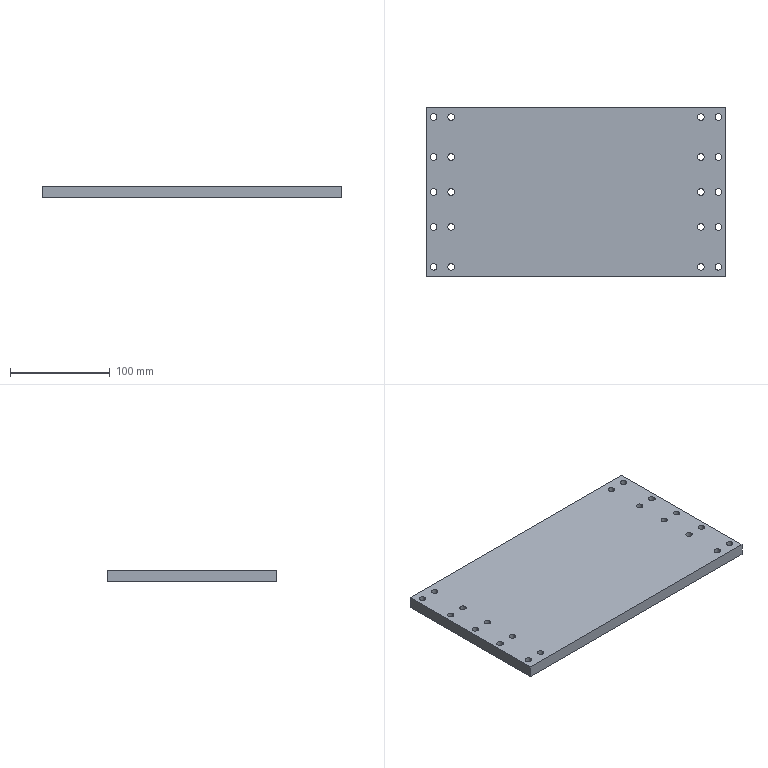Component | SolidWorks | JL001-04-01-001-1 | 1 solid | 76 faces | box 300 x 170 x 12 mm | volume 599777 mm3 | cylinder 60 | plane 16 | commonest cylinder face diameters 6.5 x20 11 x20 6.6 x20
build123d program:
from build123d import *

# Parameters (mm, degrees)
SKETCH1_W                                            = 300
SKETCH1_H                                            = 170
BOSS_EXTRUDE1_DEPTH                                  = 12
HOLE_SIZE_ACCORDING_TO_TYPE_1_OF_HEXAGON_D           = 6.6
HOLE_SIZE_ACCORDING_TO_TYPE_1_OF_HEXAGON_CBORE_D     = 11
HOLE_SIZE_ACCORDING_TO_TYPE_1_OF_HEXAGON_CBORE_DEPTH = 6.8
F_6_5_6_5_DIAMETER_HOLE1_D                           = 6.5


with BuildPart() as part:
    # Sketch1 → Boss-Extrude1 (new body)
    with BuildSketch(Plane.XY):
        Rectangle(SKETCH1_W, SKETCH1_H)
    extrude(amount=BOSS_EXTRUDE1_DEPTH)

    # Hole Size_According to_Type 1 of Hexagon (through all)
    with Locations(Plane(origin=(0, 0, 0), x_dir=(1, 0, 0), z_dir=(0, 0, -1))):
        with Locations((-142.5, -75), (-142.5, 0), (-142.5, 75), (142.5, -75), (142.5, 0), (142.5, 75), (142.5, -35), (142.5, 35), (-142.5, -35), (-142.5, 35)):
            CounterBoreHole(HOLE_SIZE_ACCORDING_TO_TYPE_1_OF_HEXAGON_D / 2, HOLE_SIZE_ACCORDING_TO_TYPE_1_OF_HEXAGON_CBORE_D / 2, HOLE_SIZE_ACCORDING_TO_TYPE_1_OF_HEXAGON_CBORE_DEPTH)

    # 6.5 _6.5_ Diameter Hole1 (through all)
    with Locations(Plane.XY.offset(12)):
        with Locations((-125, 75), (-125, 0), (-125, -75), (125, 75), (125, 0), (125, -75), (-125, 35), (-125, -35), (125, 35), (125, -35)):
            Hole(F_6_5_6_5_DIAMETER_HOLE1_D / 2)


solid = part.part